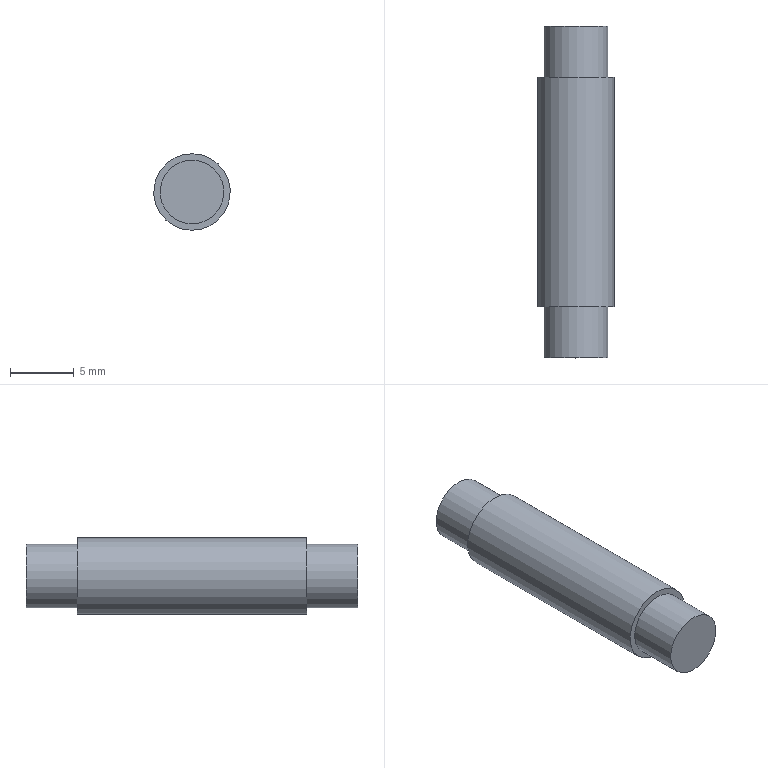Component | NX | LINK_PIN | 1 solid | 7 faces | volume 666 mm3 | plane 4 | cylinder 3 | commonest cylinder face diameters 5 x2 6 x1